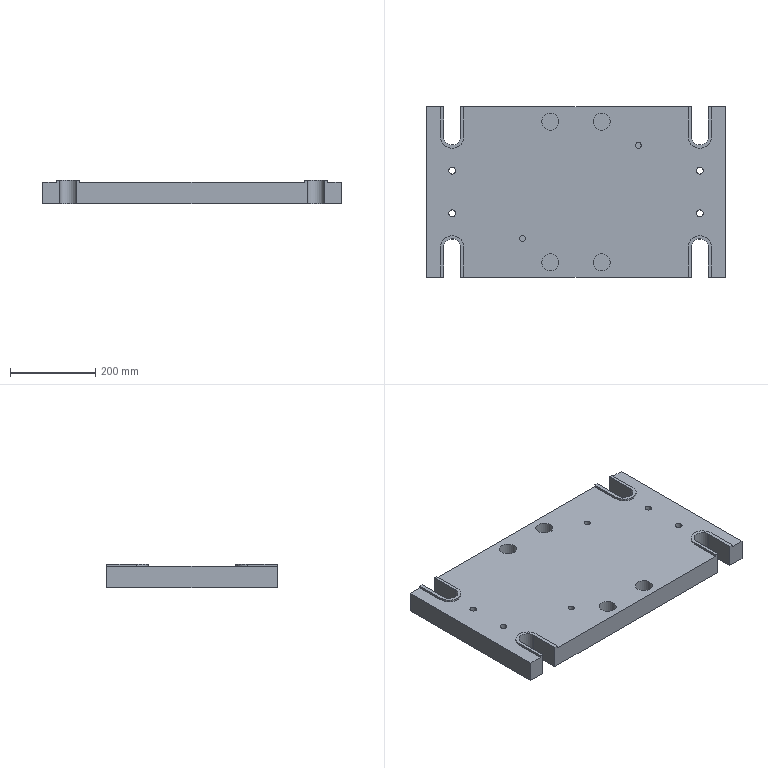Component | NX | FIXTURE_BASE | 1 solid | 62 faces | volume 13102741 mm3 | plane 40 | cylinder 22 | commonest cylinder face diameters 40 x8 16 x4 55 x4 30 x4 14 x2